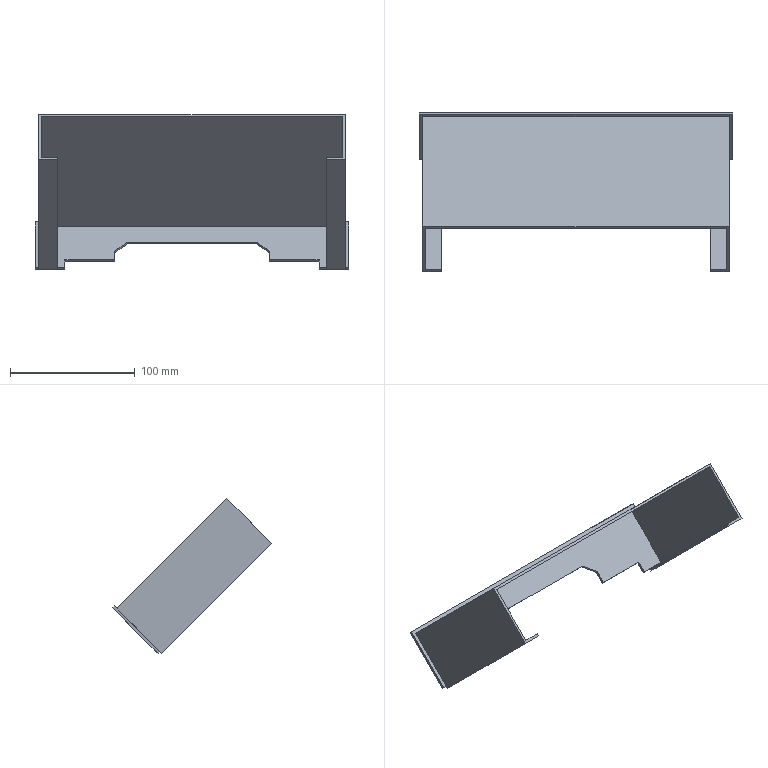Component | SolidWorks | Section3-1 | 2 solids | 30 faces | box 252 x 127.99 x 124.45 mm | volume 110276 mm3 | plane 30
build123d program:
from build123d import *

# Parameters (mm, degrees)
EXTRUDE_THIN1_DEPTH = 125
BOSS_EXTRUDE1_DEPTH = 2


with BuildPart() as part:
    # Sketch1 → Extrude-Thin1 (new body)
    with BuildSketch(Plane.XY):
        Polygon((-42.5, -44), (-57.5, -44), (-57.5, 7), (188.5, 7), (188.5, -44), (173.5, -44), (173.5, -42), (186.5, -42), (186.5, 5), (-55.5, 5), (-55.5, -42), (-42.5, -42), align=None)
    extrude(amount=EXTRUDE_THIN1_DEPTH)


with BuildPart() as body_2:
    # Sketch3 → Boss-Extrude1 (new body)
    with BuildSketch(Plane(origin=(0, 0, 0), x_dir=(-1, 0, 0), z_dir=(0, 0, -1))):
        Polygon((-167.5, -42), (-191.5, -42), (-191.5, 10), (60.5, 10), (60.5, -42), (36.5, -42), (36.5, -33), (-3.5, -33), (-3.5, -23), (-13.5, -13), (-117.5, -13), (-127.5, -23), (-127.5, -33), (-167.5, -33), align=None)
    extrude(amount=BOSS_EXTRUDE1_DEPTH)


solid = Compound([part.part, body_2.part])

# Placed as in the assembly
solid = solid.moved(Location((53.324, -324.22, 131.269), (45, 0, 0)))
STEP:
#1=COLOUR_RGB('',0.7922,0.8196,0.9333);
#2=FILL_AREA_STYLE_COLOUR('',#1);
#3=FILL_AREA_STYLE('',(#2));
#4=SURFACE_STYLE_FILL_AREA(#3);
#5=SURFACE_SIDE_STYLE('',(#4));
#6=SURFACE_STYLE_USAGE(.BOTH.,#5);
#7=PRESENTATION_STYLE_ASSIGNMENT((#6));
#8=CARTESIAN_POINT('',(8.694,-13.934,3.999));
#9=VERTEX_POINT('',#8);
#10=CARTESIAN_POINT('',(8.694,-13.683,4.249));
#11=VERTEX_POINT('',#10);
#12=CARTESIAN_POINT('',(8.694,-13.683,4.249));
#13=DIRECTION('',(-0.,0.7071,0.7071));
#14=VECTOR('',#13,39.37);
#15=LINE('',#12,#14);
#16=EDGE_CURVE('',#9,#11,#15,.T.);
#17=ORIENTED_EDGE('',*,*,#16,.T.);
#18=CARTESIAN_POINT('',(8.694,-13.628,4.194));
#19=VERTEX_POINT('',#18);
#20=CARTESIAN_POINT('',(8.694,-13.628,4.194));
#21=DIRECTION('',(0.,-0.7071,0.7071));
#22=VECTOR('',#21,39.37);
#23=LINE('',#20,#22);
#24=EDGE_CURVE('',#19,#11,#23,.T.);
#25=ORIENTED_EDGE('',*,*,#24,.F.);
#26=CARTESIAN_POINT('',(8.694,-13.878,3.943));
#27=VERTEX_POINT('',#26);
#28=CARTESIAN_POINT('',(8.694,-13.628,4.194));
#29=DIRECTION('',(-0.,0.7071,0.7071));
#30=VECTOR('',#29,39.37);
#31=LINE('',#28,#30);
#32=EDGE_CURVE('',#27,#19,#31,.T.);
#33=ORIENTED_EDGE('',*,*,#32,.F.);
#34=CARTESIAN_POINT('',(8.694,-13.878,3.943));
#35=DIRECTION('',(0.,-0.7071,0.7071));
#36=VECTOR('',#35,39.37);
#37=LINE('',#34,#36);
#38=EDGE_CURVE('',#27,#9,#37,.T.);
#39=ORIENTED_EDGE('',*,*,#38,.T.);
#40=EDGE_LOOP('',(#17,#25,#33,#39));
#41=FACE_OUTER_BOUND('',#40,.T.);
#42=CARTESIAN_POINT('',(8.694,-13.628,4.194));
#43=DIRECTION('',(1.,0.,-0.));
#44=DIRECTION('',(-0.,0.7071,-0.7071));
#45=AXIS2_PLACEMENT_3D('',#42,#43,#44);
#46=PLANE('',#45);
#47=ADVANCED_FACE('',(#41),#46,.F.);
#48=CARTESIAN_POINT('',(7.119,-13.683,4.249));
#49=VERTEX_POINT('',#48);
#50=CARTESIAN_POINT('',(7.119,-13.683,4.249));
#51=DIRECTION('',(-1.,-0.,0.));
#52=VECTOR('',#51,39.37);
#53=LINE('',#50,#52);
#54=EDGE_CURVE('',#11,#49,#53,.T.);
#55=ORIENTED_EDGE('',*,*,#54,.T.);
#56=CARTESIAN_POINT('',(7.119,-13.628,4.194));
#57=VERTEX_POINT('',#56);
#58=CARTESIAN_POINT('',(7.119,-13.628,4.194));
#59=DIRECTION('',(0.,-0.7071,0.7071));
#60=VECTOR('',#59,39.37);
#61=LINE('',#58,#60);
#62=EDGE_CURVE('',#57,#49,#61,.T.);
#63=ORIENTED_EDGE('',*,*,#62,.F.);
#64=CARTESIAN_POINT('',(7.119,-13.628,4.194));
#65=DIRECTION('',(-1.,-0.,0.));
#66=VECTOR('',#65,39.37);
#67=LINE('',#64,#66);
#68=EDGE_CURVE('',#19,#57,#67,.T.);
#69=ORIENTED_EDGE('',*,*,#68,.F.);
#70=ORIENTED_EDGE('',*,*,#24,.T.);
#71=EDGE_LOOP('',(#55,#63,#69,#70));
#72=FACE_OUTER_BOUND('',#71,.T.);
#73=CARTESIAN_POINT('',(7.119,-13.628,4.194));
#74=DIRECTION('',(-0.,0.7071,0.7071));
#75=DIRECTION('',(0.,-0.7071,0.7071));
#76=AXIS2_PLACEMENT_3D('',#73,#74,#75);
#77=PLANE('',#76);
#78=ADVANCED_FACE('',(#72),#77,.F.);
#79=CARTESIAN_POINT('',(7.119,-13.405,4.528));
#80=VERTEX_POINT('',#79);
#81=CARTESIAN_POINT('',(7.119,-13.405,4.528));
#82=DIRECTION('',(0.,0.7071,0.7071));
#83=VECTOR('',#82,39.37);
#84=LINE('',#81,#83);
#85=EDGE_CURVE('',#49,#80,#84,.T.);
#86=ORIENTED_EDGE('',*,*,#85,.T.);
#87=CARTESIAN_POINT('',(7.119,-13.349,4.472));
#88=VERTEX_POINT('',#87);
#89=CARTESIAN_POINT('',(7.119,-13.349,4.472));
#90=DIRECTION('',(0.,-0.7071,0.7071));
#91=VECTOR('',#90,39.37);
#92=LINE('',#89,#91);
#93=EDGE_CURVE('',#88,#80,#92,.T.);
#94=ORIENTED_EDGE('',*,*,#93,.F.);
#95=CARTESIAN_POINT('',(7.119,-13.349,4.472));
#96=DIRECTION('',(0.,0.7071,0.7071));
#97=VECTOR('',#96,39.37);
#98=LINE('',#95,#97);
#99=EDGE_CURVE('',#57,#88,#98,.T.);
#100=ORIENTED_EDGE('',*,*,#99,.F.);
#101=ORIENTED_EDGE('',*,*,#62,.T.);
#102=EDGE_LOOP('',(#86,#94,#100,#101));
#103=FACE_OUTER_BOUND('',#102,.T.);
#104=CARTESIAN_POINT('',(7.119,-13.349,4.472));
#105=DIRECTION('',(1.,-0.,-0.));
#106=DIRECTION('',(0.,0.7071,0.7071));
#107=AXIS2_PLACEMENT_3D('',#104,#105,#106);
#108=PLANE('',#107);
#109=ADVANCED_FACE('',(#103),#108,.F.);
#110=CARTESIAN_POINT('',(6.725,-13.126,4.806));
#111=VERTEX_POINT('',#110);
#112=CARTESIAN_POINT('',(6.725,-13.126,4.806));
#113=DIRECTION('',(-0.7071,0.5,0.5));
#114=VECTOR('',#113,39.37);
#115=LINE('',#112,#114);
#116=EDGE_CURVE('',#80,#111,#115,.T.);
#117=ORIENTED_EDGE('',*,*,#116,.T.);
#118=CARTESIAN_POINT('',(6.725,-13.071,4.751));
#119=VERTEX_POINT('',#118);
#120=CARTESIAN_POINT('',(6.725,-13.071,4.751));
#121=DIRECTION('',(0.,-0.7071,0.7071));
#122=VECTOR('',#121,39.37);
#123=LINE('',#120,#122);
#124=EDGE_CURVE('',#119,#111,#123,.T.);
#125=ORIENTED_EDGE('',*,*,#124,.F.);
#126=CARTESIAN_POINT('',(6.725,-13.071,4.751));
#127=DIRECTION('',(-0.7071,0.5,0.5));
#128=VECTOR('',#127,39.37);
#129=LINE('',#126,#128);
#130=EDGE_CURVE('',#88,#119,#129,.T.);
#131=ORIENTED_EDGE('',*,*,#130,.F.);
#132=ORIENTED_EDGE('',*,*,#93,.T.);
#133=EDGE_LOOP('',(#117,#125,#131,#132));
#134=FACE_OUTER_BOUND('',#133,.T.);
#135=CARTESIAN_POINT('',(6.725,-13.071,4.751));
#136=DIRECTION('',(0.7071,0.5,0.5));
#137=DIRECTION('',(-0.7071,0.5,0.5));
#138=AXIS2_PLACEMENT_3D('',#135,#136,#137);
#139=PLANE('',#138);
#140=ADVANCED_FACE('',(#134),#139,.F.);
#141=CARTESIAN_POINT('',(2.631,-13.126,4.806));
#142=VERTEX_POINT('',#141);
#143=CARTESIAN_POINT('',(2.631,-13.126,4.806));
#144=DIRECTION('',(-1.,-0.,0.));
#145=VECTOR('',#144,39.37);
#146=LINE('',#143,#145);
#147=EDGE_CURVE('',#111,#142,#146,.T.);
#148=ORIENTED_EDGE('',*,*,#147,.T.);
#149=CARTESIAN_POINT('',(2.631,-13.071,4.751));
#150=VERTEX_POINT('',#149);
#151=CARTESIAN_POINT('',(2.631,-13.071,4.751));
#152=DIRECTION('',(0.,-0.7071,0.7071));
#153=VECTOR('',#152,39.37);
#154=LINE('',#151,#153);
#155=EDGE_CURVE('',#150,#142,#154,.T.);
#156=ORIENTED_EDGE('',*,*,#155,.F.);
#157=CARTESIAN_POINT('',(2.631,-13.071,4.751));
#158=DIRECTION('',(-1.,-0.,0.));
#159=VECTOR('',#158,39.37);
#160=LINE('',#157,#159);
#161=EDGE_CURVE('',#119,#150,#160,.T.);
#162=ORIENTED_EDGE('',*,*,#161,.F.);
#163=ORIENTED_EDGE('',*,*,#124,.T.);
#164=EDGE_LOOP('',(#148,#156,#162,#163));
#165=FACE_OUTER_BOUND('',#164,.T.);
#166=CARTESIAN_POINT('',(2.631,-13.071,4.751));
#167=DIRECTION('',(0.,0.7071,0.7071));
#168=DIRECTION('',(-1.,-0.,0.));
#169=AXIS2_PLACEMENT_3D('',#166,#167,#168);
#170=PLANE('',#169);
#171=ADVANCED_FACE('',(#165),#170,.F.);
#172=CARTESIAN_POINT('',(2.237,-13.405,4.528));
#173=VERTEX_POINT('',#172);
#174=CARTESIAN_POINT('',(2.237,-13.405,4.528));
#175=DIRECTION('',(-0.7071,-0.5,-0.5));
#176=VECTOR('',#175,39.37);
#177=LINE('',#174,#176);
#178=EDGE_CURVE('',#142,#173,#177,.T.);
#179=ORIENTED_EDGE('',*,*,#178,.T.);
#180=CARTESIAN_POINT('',(2.237,-13.349,4.472));
#181=VERTEX_POINT('',#180);
#182=CARTESIAN_POINT('',(2.237,-13.349,4.472));
#183=DIRECTION('',(0.,-0.7071,0.7071));
#184=VECTOR('',#183,39.37);
#185=LINE('',#182,#184);
#186=EDGE_CURVE('',#181,#173,#185,.T.);
#187=ORIENTED_EDGE('',*,*,#186,.F.);
#188=CARTESIAN_POINT('',(2.237,-13.349,4.472));
#189=DIRECTION('',(-0.7071,-0.5,-0.5));
#190=VECTOR('',#189,39.37);
#191=LINE('',#188,#190);
#192=EDGE_CURVE('',#150,#181,#191,.T.);
#193=ORIENTED_EDGE('',*,*,#192,.F.);
#194=ORIENTED_EDGE('',*,*,#155,.T.);
#195=EDGE_LOOP('',(#179,#187,#193,#194));
#196=FACE_OUTER_BOUND('',#195,.T.);
#197=CARTESIAN_POINT('',(2.237,-13.349,4.472));
#198=DIRECTION('',(-0.7071,0.5,0.5));
#199=DIRECTION('',(-0.7071,-0.5,-0.5));
#200=AXIS2_PLACEMENT_3D('',#197,#198,#199);
#201=PLANE('',#200);
#202=ADVANCED_FACE('',(#196),#201,.F.);
#203=CARTESIAN_POINT('',(2.237,-13.683,4.249));
#204=VERTEX_POINT('',#203);
#205=CARTESIAN_POINT('',(2.237,-13.683,4.249));
#206=DIRECTION('',(-0.,-0.7071,-0.7071));
#207=VECTOR('',#206,39.37);
#208=LINE('',#205,#207);
#209=EDGE_CURVE('',#173,#204,#208,.T.);
#210=ORIENTED_EDGE('',*,*,#209,.T.);
#211=CARTESIAN_POINT('',(2.237,-13.628,4.194));
#212=VERTEX_POINT('',#211);
#213=CARTESIAN_POINT('',(2.237,-13.628,4.194));
#214=DIRECTION('',(0.,-0.7071,0.7071));
#215=VECTOR('',#214,39.37);
#216=LINE('',#213,#215);
#217=EDGE_CURVE('',#212,#204,#216,.T.);
#218=ORIENTED_EDGE('',*,*,#217,.F.);
#219=CARTESIAN_POINT('',(2.237,-13.628,4.194));
#220=DIRECTION('',(-0.,-0.7071,-0.7071));
#221=VECTOR('',#220,39.37);
#222=LINE('',#219,#221);
#223=EDGE_CURVE('',#181,#212,#222,.T.);
#224=ORIENTED_EDGE('',*,*,#223,.F.);
#225=ORIENTED_EDGE('',*,*,#186,.T.);
#226=EDGE_LOOP('',(#210,#218,#224,#225));
#227=FACE_OUTER_BOUND('',#226,.T.);
#228=CARTESIAN_POINT('',(2.237,-13.628,4.194));
#229=DIRECTION('',(-1.,0.,0.));
#230=DIRECTION('',(-0.,-0.7071,-0.7071));
#231=AXIS2_PLACEMENT_3D('',#228,#229,#230);
#232=PLANE('',#231);
#233=ADVANCED_FACE('',(#227),#232,.F.);
#234=CARTESIAN_POINT('',(0.6624,-13.683,4.249));
#235=VERTEX_POINT('',#234);
#236=CARTESIAN_POINT('',(0.6624,-13.683,4.249));
#237=DIRECTION('',(-1.,-0.,0.));
#238=VECTOR('',#237,39.37);
#239=LINE('',#236,#238);
#240=EDGE_CURVE('',#204,#235,#239,.T.);
#241=ORIENTED_EDGE('',*,*,#240,.T.);
#242=CARTESIAN_POINT('',(0.6624,-13.628,4.194));
#243=VERTEX_POINT('',#242);
#244=CARTESIAN_POINT('',(0.6624,-13.628,4.194));
#245=DIRECTION('',(0.,-0.7071,0.7071));
#246=VECTOR('',#245,39.37);
#247=LINE('',#244,#246);
#248=EDGE_CURVE('',#243,#235,#247,.T.);
#249=ORIENTED_EDGE('',*,*,#248,.F.);
#250=CARTESIAN_POINT('',(0.6624,-13.628,4.194));
#251=DIRECTION('',(-1.,-0.,0.));
#252=VECTOR('',#251,39.37);
#253=LINE('',#250,#252);
#254=EDGE_CURVE('',#212,#243,#253,.T.);
#255=ORIENTED_EDGE('',*,*,#254,.F.);
#256=ORIENTED_EDGE('',*,*,#217,.T.);
#257=EDGE_LOOP('',(#241,#249,#255,#256));
#258=FACE_OUTER_BOUND('',#257,.T.);
#259=CARTESIAN_POINT('',(0.6624,-13.628,4.194));
#260=DIRECTION('',(0.,0.7071,0.7071));
#261=DIRECTION('',(-1.,-0.,0.));
#262=AXIS2_PLACEMENT_3D('',#259,#260,#261);
#263=PLANE('',#262);
#264=ADVANCED_FACE('',(#258),#263,.F.);
#265=CARTESIAN_POINT('',(0.6624,-13.934,3.999));
#266=VERTEX_POINT('',#265);
#267=CARTESIAN_POINT('',(0.6624,-13.934,3.999));
#268=DIRECTION('',(0.,-0.7071,-0.7071));
#269=VECTOR('',#268,39.37);
#270=LINE('',#267,#269);
#271=EDGE_CURVE('',#235,#266,#270,.T.);
#272=ORIENTED_EDGE('',*,*,#271,.T.);
#273=CARTESIAN_POINT('',(0.6624,-13.878,3.943));
#274=VERTEX_POINT('',#273);
#275=CARTESIAN_POINT('',(0.6624,-13.878,3.943));
#276=DIRECTION('',(0.,-0.7071,0.7071));
#277=VECTOR('',#276,39.37);
#278=LINE('',#275,#277);
#279=EDGE_CURVE('',#274,#266,#278,.T.);
#280=ORIENTED_EDGE('',*,*,#279,.F.);
#281=CARTESIAN_POINT('',(0.6624,-13.878,3.943));
#282=DIRECTION('',(0.,-0.7071,-0.7071));
#283=VECTOR('',#282,39.37);
#284=LINE('',#281,#283);
#285=EDGE_CURVE('',#243,#274,#284,.T.);
#286=ORIENTED_EDGE('',*,*,#285,.F.);
#287=ORIENTED_EDGE('',*,*,#248,.T.);
#288=EDGE_LOOP('',(#272,#280,#286,#287));
#289=FACE_OUTER_BOUND('',#288,.T.);
#290=CARTESIAN_POINT('',(0.6624,-13.878,3.943));
#291=DIRECTION('',(-1.,-0.,0.));
#292=DIRECTION('',(0.,-0.7071,0.7071));
#293=AXIS2_PLACEMENT_3D('',#290,#291,#292);
#294=PLANE('',#293);
#295=ADVANCED_FACE('',(#289),#294,.F.);
#296=CARTESIAN_POINT('',(-0.2825,-13.934,3.999));
#297=VERTEX_POINT('',#296);
#298=CARTESIAN_POINT('',(-0.2825,-13.934,3.999));
#299=DIRECTION('',(-1.,-0.,0.));
#300=VECTOR('',#299,39.37);
#301=LINE('',#298,#300);
#302=EDGE_CURVE('',#266,#297,#301,.T.);
#303=ORIENTED_EDGE('',*,*,#302,.T.);
#304=CARTESIAN_POINT('',(-0.2825,-13.878,3.943));
#305=VERTEX_POINT('',#304);
#306=CARTESIAN_POINT('',(-0.2825,-13.878,3.943));
#307=DIRECTION('',(0.,-0.7071,0.7071));
#308=VECTOR('',#307,39.37);
#309=LINE('',#306,#308);
#310=EDGE_CURVE('',#305,#297,#309,.T.);
#311=ORIENTED_EDGE('',*,*,#310,.F.);
#312=CARTESIAN_POINT('',(-0.2825,-13.878,3.943));
#313=DIRECTION('',(-1.,-0.,0.));
#314=VECTOR('',#313,39.37);
#315=LINE('',#312,#314);
#316=EDGE_CURVE('',#274,#305,#315,.T.);
#317=ORIENTED_EDGE('',*,*,#316,.F.);
#318=ORIENTED_EDGE('',*,*,#279,.T.);
#319=EDGE_LOOP('',(#303,#311,#317,#318));
#320=FACE_OUTER_BOUND('',#319,.T.);
#321=CARTESIAN_POINT('',(-0.2825,-13.878,3.943));
#322=DIRECTION('',(-0.,0.7071,0.7071));
#323=DIRECTION('',(0.,-0.7071,0.7071));
#324=AXIS2_PLACEMENT_3D('',#321,#322,#323);
#325=PLANE('',#324);
#326=ADVANCED_FACE('',(#320),#325,.F.);
#327=CARTESIAN_POINT('',(-0.2825,-12.486,5.446));
#328=VERTEX_POINT('',#327);
#329=CARTESIAN_POINT('',(-0.2825,-12.486,5.446));
#330=DIRECTION('',(0.,0.7071,0.7071));
#331=VECTOR('',#330,39.37);
#332=LINE('',#329,#331);
#333=EDGE_CURVE('',#297,#328,#332,.T.);
#334=ORIENTED_EDGE('',*,*,#333,.T.);
#335=CARTESIAN_POINT('',(-0.2825,-12.431,5.391));
#336=VERTEX_POINT('',#335);
#337=CARTESIAN_POINT('',(-0.2825,-12.431,5.391));
#338=DIRECTION('',(0.,-0.7071,0.7071));
#339=VECTOR('',#338,39.37);
#340=LINE('',#337,#339);
#341=EDGE_CURVE('',#336,#328,#340,.T.);
#342=ORIENTED_EDGE('',*,*,#341,.F.);
#343=CARTESIAN_POINT('',(-0.2825,-12.431,5.391));
#344=DIRECTION('',(0.,0.7071,0.7071));
#345=VECTOR('',#344,39.37);
#346=LINE('',#343,#345);
#347=EDGE_CURVE('',#305,#336,#346,.T.);
#348=ORIENTED_EDGE('',*,*,#347,.F.);
#349=ORIENTED_EDGE('',*,*,#310,.T.);
#350=EDGE_LOOP('',(#334,#342,#348,#349));
#351=FACE_OUTER_BOUND('',#350,.T.);
#352=CARTESIAN_POINT('',(-0.2825,-12.431,5.391));
#353=DIRECTION('',(1.,0.,-0.));
#354=DIRECTION('',(0.,0.7071,0.7071));
#355=AXIS2_PLACEMENT_3D('',#352,#353,#354);
#356=PLANE('',#355);
#357=ADVANCED_FACE('',(#351),#356,.F.);
#358=CARTESIAN_POINT('',(9.639,-12.486,5.446));
#359=VERTEX_POINT('',#358);
#360=CARTESIAN_POINT('',(9.639,-12.486,5.446));
#361=DIRECTION('',(1.,0.,-0.));
#362=VECTOR('',#361,39.37);
#363=LINE('',#360,#362);
#364=EDGE_CURVE('',#328,#359,#363,.T.);
#365=ORIENTED_EDGE('',*,*,#364,.T.);
#366=CARTESIAN_POINT('',(9.639,-12.431,5.391));
#367=VERTEX_POINT('',#366);
#368=CARTESIAN_POINT('',(9.639,-12.431,5.391));
#369=DIRECTION('',(0.,-0.7071,0.7071));
#370=VECTOR('',#369,39.37);
#371=LINE('',#368,#370);
#372=EDGE_CURVE('',#367,#359,#371,.T.);
#373=ORIENTED_EDGE('',*,*,#372,.F.);
#374=CARTESIAN_POINT('',(9.639,-12.431,5.391));
#375=DIRECTION('',(1.,0.,-0.));
#376=VECTOR('',#375,39.37);
#377=LINE('',#374,#376);
#378=EDGE_CURVE('',#336,#367,#377,.T.);
#379=ORIENTED_EDGE('',*,*,#378,.F.);
#380=ORIENTED_EDGE('',*,*,#341,.T.);
#381=EDGE_LOOP('',(#365,#373,#379,#380));
#382=FACE_OUTER_BOUND('',#381,.T.);
#383=CARTESIAN_POINT('',(9.639,-12.431,5.391));
#384=DIRECTION('',(0.,-0.7071,-0.7071));
#385=DIRECTION('',(-0.,0.7071,-0.7071));
#386=AXIS2_PLACEMENT_3D('',#383,#384,#385);
#387=PLANE('',#386);
#388=ADVANCED_FACE('',(#382),#387,.F.);
#389=CARTESIAN_POINT('',(9.639,-13.934,3.999));
#390=VERTEX_POINT('',#389);
#391=CARTESIAN_POINT('',(9.639,-13.934,3.999));
#392=DIRECTION('',(0.,-0.7071,-0.7071));
#393=VECTOR('',#392,39.37);
#394=LINE('',#391,#393);
#395=EDGE_CURVE('',#359,#390,#394,.T.);
#396=ORIENTED_EDGE('',*,*,#395,.T.);
#397=CARTESIAN_POINT('',(9.639,-13.878,3.943));
#398=VERTEX_POINT('',#397);
#399=CARTESIAN_POINT('',(9.639,-13.878,3.943));
#400=DIRECTION('',(0.,-0.7071,0.7071));
#401=VECTOR('',#400,39.37);
#402=LINE('',#399,#401);
#403=EDGE_CURVE('',#398,#390,#402,.T.);
#404=ORIENTED_EDGE('',*,*,#403,.F.);
#405=CARTESIAN_POINT('',(9.639,-13.878,3.943));
#406=DIRECTION('',(0.,-0.7071,-0.7071));
#407=VECTOR('',#406,39.37);
#408=LINE('',#405,#407);
#409=EDGE_CURVE('',#367,#398,#408,.T.);
#410=ORIENTED_EDGE('',*,*,#409,.F.);
#411=ORIENTED_EDGE('',*,*,#372,.T.);
#412=EDGE_LOOP('',(#396,#404,#410,#411));
#413=FACE_OUTER_BOUND('',#412,.T.);
#414=CARTESIAN_POINT('',(9.639,-13.878,3.943));
#415=DIRECTION('',(-1.,-0.,0.));
#416=DIRECTION('',(0.,-0.7071,0.7071));
#417=AXIS2_PLACEMENT_3D('',#414,#415,#416);
#418=PLANE('',#417);
#419=ADVANCED_FACE('',(#413),#418,.F.);
#420=CARTESIAN_POINT('',(8.694,-13.934,3.999));
#421=DIRECTION('',(-1.,-0.,-0.));
#422=VECTOR('',#421,39.37);
#423=LINE('',#420,#422);
#424=EDGE_CURVE('',#390,#9,#423,.T.);
#425=ORIENTED_EDGE('',*,*,#424,.T.);
#426=ORIENTED_EDGE('',*,*,#38,.F.);
#427=CARTESIAN_POINT('',(8.694,-13.878,3.943));
#428=DIRECTION('',(-1.,-0.,-0.));
#429=VECTOR('',#428,39.37);
#430=LINE('',#427,#429);
#431=EDGE_CURVE('',#398,#27,#430,.T.);
#432=ORIENTED_EDGE('',*,*,#431,.F.);
#433=ORIENTED_EDGE('',*,*,#403,.T.);
#434=EDGE_LOOP('',(#425,#426,#432,#433));
#435=FACE_OUTER_BOUND('',#434,.T.);
#436=CARTESIAN_POINT('',(8.694,-13.878,3.943));
#437=DIRECTION('',(-0.,0.7071,0.7071));
#438=DIRECTION('',(-1.,-0.,-0.));
#439=AXIS2_PLACEMENT_3D('',#436,#437,#438);
#440=PLANE('',#439);
#441=ADVANCED_FACE('',(#435),#440,.F.);
#442=ORIENTED_EDGE('',*,*,#32,.T.);
#443=ORIENTED_EDGE('',*,*,#68,.T.);
#444=ORIENTED_EDGE('',*,*,#99,.T.);
#445=ORIENTED_EDGE('',*,*,#130,.T.);
#446=ORIENTED_EDGE('',*,*,#161,.T.);
#447=ORIENTED_EDGE('',*,*,#192,.T.);
#448=ORIENTED_EDGE('',*,*,#223,.T.);
#449=ORIENTED_EDGE('',*,*,#254,.T.);
#450=ORIENTED_EDGE('',*,*,#285,.T.);
#451=ORIENTED_EDGE('',*,*,#316,.T.);
#452=ORIENTED_EDGE('',*,*,#347,.T.);
#453=ORIENTED_EDGE('',*,*,#378,.T.);
#454=ORIENTED_EDGE('',*,*,#409,.T.);
#455=ORIENTED_EDGE('',*,*,#431,.T.);
#456=EDGE_LOOP('',(#442,#443,#444,#445,#446,#447,#448,#449,#450,#451,#452,#453,#454,#455));
#457=FACE_OUTER_BOUND('',#456,.T.);
#458=CARTESIAN_POINT('',(2.099,-12.709,5.112));
#459=DIRECTION('',(0.,-0.7071,0.7071));
#460=DIRECTION('',(1.,0.,-0.));
#461=AXIS2_PLACEMENT_3D('',#458,#459,#460);
#462=PLANE('',#461);
#463=ADVANCED_FACE('',(#457),#462,.F.);
#464=ORIENTED_EDGE('',*,*,#16,.F.);
#465=ORIENTED_EDGE('',*,*,#424,.F.);
#466=ORIENTED_EDGE('',*,*,#395,.F.);
#467=ORIENTED_EDGE('',*,*,#364,.F.);
#468=ORIENTED_EDGE('',*,*,#333,.F.);
#469=ORIENTED_EDGE('',*,*,#302,.F.);
#470=ORIENTED_EDGE('',*,*,#271,.F.);
#471=ORIENTED_EDGE('',*,*,#240,.F.);
#472=ORIENTED_EDGE('',*,*,#209,.F.);
#473=ORIENTED_EDGE('',*,*,#178,.F.);
#474=ORIENTED_EDGE('',*,*,#147,.F.);
#475=ORIENTED_EDGE('',*,*,#116,.F.);
#476=ORIENTED_EDGE('',*,*,#85,.F.);
#477=ORIENTED_EDGE('',*,*,#54,.F.);
#478=EDGE_LOOP('',(#464,#465,#466,#467,#468,#469,#470,#471,#472,#473,#474,#475,#476,#477));
#479=FACE_OUTER_BOUND('',#478,.T.);
#480=CARTESIAN_POINT('',(2.099,-12.765,5.168));
#481=DIRECTION('',(0.,-0.7071,0.7071));
#482=DIRECTION('',(1.,0.,-0.));
#483=AXIS2_PLACEMENT_3D('',#480,#481,#482);
#484=PLANE('',#483);
#485=ADVANCED_FACE('',(#479),#484,.T.);
#486=CLOSED_SHELL('',(#47,#78,#109,#140,#171,#202,#233,#264,#295,#326,#357,#388,#419,#441,#463,#485));
#487=MANIFOLD_SOLID_BREP('',#486);
#488=STYLED_ITEM('',(#7),#487);
#489=(LENGTH_UNIT()NAMED_UNIT(*)SI_UNIT($,.METRE.));
#490=LENGTH_MEASURE_WITH_UNIT(LENGTH_MEASURE(0.0254),#489);
#491=DIMENSIONAL_EXPONENTS(1.,0.,0.,0.,0.,0.,0.);
#492=(CONVERSION_BASED_UNIT('',#490)LENGTH_UNIT()NAMED_UNIT(#491));
#493=UNCERTAINTY_MEASURE_WITH_UNIT(LENGTH_MEASURE(0.00001),#492,'','');
#494=(NAMED_UNIT(*)PLANE_ANGLE_UNIT()SI_UNIT($,.RADIAN.));
#495=(NAMED_UNIT(*)SI_UNIT($,.STERADIAN.)SOLID_ANGLE_UNIT());
#496=(GEOMETRIC_REPRESENTATION_CONTEXT(3)GLOBAL_UNCERTAINTY_ASSIGNED_CONTEXT((#493))GLOBAL_UNIT_ASSIGNED_CONTEXT((#492,#494,#495))REPRESENTATION_CONTEXT('',''));
#497=MECHANICAL_DESIGN_GEOMETRIC_PRESENTATION_REPRESENTATION('',(#488),#496);
#498=PRESENTATION_LAYER_ASSIGNMENT('','',(#488));
#499=CARTESIAN_POINT('',(9.442,-13.934,3.999));
#500=VERTEX_POINT('',#499);
#501=CARTESIAN_POINT('',(8.93,-13.934,3.999));
#502=VERTEX_POINT('',#501);
#503=CARTESIAN_POINT('',(9.521,-13.934,3.999));
#504=DIRECTION('',(-1.,-0.,-0.));
#505=VECTOR('',#504,39.37);
#506=LINE('',#503,#505);
#507=EDGE_CURVE('',#500,#502,#506,.T.);
#508=ORIENTED_EDGE('',*,*,#507,.T.);
#509=CARTESIAN_POINT('',(8.93,-17.414,7.479));
#510=VERTEX_POINT('',#509);
#511=CARTESIAN_POINT('',(8.93,-17.414,7.479));
#512=DIRECTION('',(-0.,0.7071,-0.7071));
#513=VECTOR('',#512,39.37);
#514=LINE('',#511,#513);
#515=EDGE_CURVE('',#510,#502,#514,.T.);
#516=ORIENTED_EDGE('',*,*,#515,.F.);
#517=CARTESIAN_POINT('',(9.442,-17.414,7.479));
#518=VERTEX_POINT('',#517);
#519=CARTESIAN_POINT('',(9.521,-17.414,7.479));
#520=DIRECTION('',(-1.,-0.,-0.));
#521=VECTOR('',#520,39.37);
#522=LINE('',#519,#521);
#523=EDGE_CURVE('',#518,#510,#522,.T.);
#524=ORIENTED_EDGE('',*,*,#523,.F.);
#525=CARTESIAN_POINT('',(9.442,-17.414,7.479));
#526=DIRECTION('',(-0.,0.7071,-0.7071));
#527=VECTOR('',#526,39.37);
#528=LINE('',#525,#527);
#529=EDGE_CURVE('',#518,#500,#528,.T.);
#530=ORIENTED_EDGE('',*,*,#529,.T.);
#531=EDGE_LOOP('',(#508,#516,#524,#530));
#532=FACE_OUTER_BOUND('',#531,.T.);
#533=CARTESIAN_POINT('',(9.521,-17.414,7.479));
#534=DIRECTION('',(0.,-0.7071,-0.7071));
#535=DIRECTION('',(1.,0.,0.));
#536=AXIS2_PLACEMENT_3D('',#533,#534,#535);
#537=PLANE('',#536);
#538=ADVANCED_FACE('',(#532),#537,.F.);
#539=CARTESIAN_POINT('',(8.93,-13.989,3.943));
#540=VERTEX_POINT('',#539);
#541=CARTESIAN_POINT('',(8.93,-13.989,3.943));
#542=DIRECTION('',(-0.,0.7071,0.7071));
#543=VECTOR('',#542,39.37);
#544=LINE('',#541,#543);
#545=EDGE_CURVE('',#540,#502,#544,.T.);
#546=ORIENTED_EDGE('',*,*,#545,.F.);
#547=CARTESIAN_POINT('',(8.93,-17.469,7.423));
#548=VERTEX_POINT('',#547);
#549=CARTESIAN_POINT('',(8.93,-17.469,7.423));
#550=DIRECTION('',(-0.,0.7071,-0.7071));
#551=VECTOR('',#550,39.37);
#552=LINE('',#549,#551);
#553=EDGE_CURVE('',#548,#540,#552,.T.);
#554=ORIENTED_EDGE('',*,*,#553,.F.);
#555=CARTESIAN_POINT('',(8.93,-17.469,7.423));
#556=DIRECTION('',(-0.,0.7071,0.7071));
#557=VECTOR('',#556,39.37);
#558=LINE('',#555,#557);
#559=EDGE_CURVE('',#548,#510,#558,.T.);
#560=ORIENTED_EDGE('',*,*,#559,.T.);
#561=ORIENTED_EDGE('',*,*,#515,.T.);
#562=EDGE_LOOP('',(#546,#554,#560,#561));
#563=FACE_OUTER_BOUND('',#562,.T.);
#564=CARTESIAN_POINT('',(8.93,-17.469,7.423));
#565=DIRECTION('',(-1.,-0.,0.));
#566=DIRECTION('',(0.,-0.7071,0.7071));
#567=AXIS2_PLACEMENT_3D('',#564,#565,#566);
#568=PLANE('',#567);
#569=ADVANCED_FACE('',(#563),#568,.T.);
#570=CARTESIAN_POINT('',(9.521,-13.989,3.943));
#571=VERTEX_POINT('',#570);
#572=CARTESIAN_POINT('',(9.521,-13.989,3.943));
#573=DIRECTION('',(-1.,-0.,-0.));
#574=VECTOR('',#573,39.37);
#575=LINE('',#572,#574);
#576=EDGE_CURVE('',#571,#540,#575,.T.);
#577=ORIENTED_EDGE('',*,*,#576,.F.);
#578=CARTESIAN_POINT('',(9.521,-17.469,7.423));
#579=VERTEX_POINT('',#578);
#580=CARTESIAN_POINT('',(9.521,-17.469,7.423));
#581=DIRECTION('',(-0.,0.7071,-0.7071));
#582=VECTOR('',#581,39.37);
#583=LINE('',#580,#582);
#584=EDGE_CURVE('',#579,#571,#583,.T.);
#585=ORIENTED_EDGE('',*,*,#584,.F.);
#586=CARTESIAN_POINT('',(9.521,-17.469,7.423));
#587=DIRECTION('',(-1.,-0.,-0.));
#588=VECTOR('',#587,39.37);
#589=LINE('',#586,#588);
#590=EDGE_CURVE('',#579,#548,#589,.T.);
#591=ORIENTED_EDGE('',*,*,#590,.T.);
#592=ORIENTED_EDGE('',*,*,#553,.T.);
#593=EDGE_LOOP('',(#577,#585,#591,#592));
#594=FACE_OUTER_BOUND('',#593,.T.);
#595=CARTESIAN_POINT('',(9.521,-17.469,7.423));
#596=DIRECTION('',(0.,-0.7071,-0.7071));
#597=DIRECTION('',(1.,0.,0.));
#598=AXIS2_PLACEMENT_3D('',#595,#596,#597);
#599=PLANE('',#598);
#600=ADVANCED_FACE('',(#594),#599,.T.);
#601=CARTESIAN_POINT('',(9.521,-12.57,5.363));
#602=VERTEX_POINT('',#601);
#603=CARTESIAN_POINT('',(9.521,-12.57,5.363));
#604=DIRECTION('',(0.,-0.7071,-0.7071));
#605=VECTOR('',#604,39.37);
#606=LINE('',#603,#605);
#607=EDGE_CURVE('',#602,#571,#606,.T.);
#608=ORIENTED_EDGE('',*,*,#607,.F.);
#609=CARTESIAN_POINT('',(9.521,-16.05,8.843));
#610=VERTEX_POINT('',#609);
#611=CARTESIAN_POINT('',(9.521,-16.05,8.843));
#612=DIRECTION('',(-0.,0.7071,-0.7071));
#613=VECTOR('',#612,39.37);
#614=LINE('',#611,#613);
#615=EDGE_CURVE('',#610,#602,#614,.T.);
#616=ORIENTED_EDGE('',*,*,#615,.F.);
#617=CARTESIAN_POINT('',(9.521,-16.05,8.843));
#618=DIRECTION('',(0.,-0.7071,-0.7071));
#619=VECTOR('',#618,39.37);
#620=LINE('',#617,#619);
#621=EDGE_CURVE('',#610,#579,#620,.T.);
#622=ORIENTED_EDGE('',*,*,#621,.T.);
#623=ORIENTED_EDGE('',*,*,#584,.T.);
#624=EDGE_LOOP('',(#608,#616,#622,#623));
#625=FACE_OUTER_BOUND('',#624,.T.);
#626=CARTESIAN_POINT('',(9.521,-16.05,8.843));
#627=DIRECTION('',(1.,0.,0.));
#628=DIRECTION('',(-0.,0.7071,0.7071));
#629=AXIS2_PLACEMENT_3D('',#626,#627,#628);
#630=PLANE('',#629);
#631=ADVANCED_FACE('',(#625),#630,.T.);
#632=CARTESIAN_POINT('',(-0.1644,-12.57,5.363));
#633=VERTEX_POINT('',#632);
#634=CARTESIAN_POINT('',(-0.1644,-12.57,5.363));
#635=DIRECTION('',(1.,0.,-0.));
#636=VECTOR('',#635,39.37);
#637=LINE('',#634,#636);
#638=EDGE_CURVE('',#633,#602,#637,.T.);
#639=ORIENTED_EDGE('',*,*,#638,.F.);
#640=CARTESIAN_POINT('',(-0.1644,-16.05,8.843));
#641=VERTEX_POINT('',#640);
#642=CARTESIAN_POINT('',(-0.1644,-16.05,8.843));
#643=DIRECTION('',(-0.,0.7071,-0.7071));
#644=VECTOR('',#643,39.37);
#645=LINE('',#642,#644);
#646=EDGE_CURVE('',#641,#633,#645,.T.);
#647=ORIENTED_EDGE('',*,*,#646,.F.);
#648=CARTESIAN_POINT('',(-0.1644,-16.05,8.843));
#649=DIRECTION('',(1.,0.,-0.));
#650=VECTOR('',#649,39.37);
#651=LINE('',#648,#650);
#652=EDGE_CURVE('',#641,#610,#651,.T.);
#653=ORIENTED_EDGE('',*,*,#652,.T.);
#654=ORIENTED_EDGE('',*,*,#615,.T.);
#655=EDGE_LOOP('',(#639,#647,#653,#654));
#656=FACE_OUTER_BOUND('',#655,.T.);
#657=CARTESIAN_POINT('',(-0.1644,-16.05,8.843));
#658=DIRECTION('',(-0.,0.7071,0.7071));
#659=DIRECTION('',(0.,-0.7071,0.7071));
#660=AXIS2_PLACEMENT_3D('',#657,#658,#659);
#661=PLANE('',#660);
#662=ADVANCED_FACE('',(#656),#661,.T.);
#663=CARTESIAN_POINT('',(-0.1644,-13.989,3.943));
#664=VERTEX_POINT('',#663);
#665=CARTESIAN_POINT('',(-0.1644,-13.989,3.943));
#666=DIRECTION('',(-0.,0.7071,0.7071));
#667=VECTOR('',#666,39.37);
#668=LINE('',#665,#667);
#669=EDGE_CURVE('',#664,#633,#668,.T.);
#670=ORIENTED_EDGE('',*,*,#669,.F.);
#671=CARTESIAN_POINT('',(-0.1644,-17.469,7.423));
#672=VERTEX_POINT('',#671);
#673=CARTESIAN_POINT('',(-0.1644,-17.469,7.423));
#674=DIRECTION('',(-0.,0.7071,-0.7071));
#675=VECTOR('',#674,39.37);
#676=LINE('',#673,#675);
#677=EDGE_CURVE('',#672,#664,#676,.T.);
#678=ORIENTED_EDGE('',*,*,#677,.F.);
#679=CARTESIAN_POINT('',(-0.1644,-17.469,7.423));
#680=DIRECTION('',(-0.,0.7071,0.7071));
#681=VECTOR('',#680,39.37);
#682=LINE('',#679,#681);
#683=EDGE_CURVE('',#672,#641,#682,.T.);
#684=ORIENTED_EDGE('',*,*,#683,.T.);
#685=ORIENTED_EDGE('',*,*,#646,.T.);
#686=EDGE_LOOP('',(#670,#678,#684,#685));
#687=FACE_OUTER_BOUND('',#686,.T.);
#688=CARTESIAN_POINT('',(-0.1644,-17.469,7.423));
#689=DIRECTION('',(-1.,-0.,0.));
#690=DIRECTION('',(0.,-0.7071,0.7071));
#691=AXIS2_PLACEMENT_3D('',#688,#689,#690);
#692=PLANE('',#691);
#693=ADVANCED_FACE('',(#687),#692,.T.);
#694=CARTESIAN_POINT('',(0.4262,-13.989,3.943));
#695=VERTEX_POINT('',#694);
#696=CARTESIAN_POINT('',(0.4262,-13.989,3.943));
#697=DIRECTION('',(-1.,-0.,0.));
#698=VECTOR('',#697,39.37);
#699=LINE('',#696,#698);
#700=EDGE_CURVE('',#695,#664,#699,.T.);
#701=ORIENTED_EDGE('',*,*,#700,.F.);
#702=CARTESIAN_POINT('',(0.4262,-17.469,7.423));
#703=VERTEX_POINT('',#702);
#704=CARTESIAN_POINT('',(0.4262,-17.469,7.423));
#705=DIRECTION('',(-0.,0.7071,-0.7071));
#706=VECTOR('',#705,39.37);
#707=LINE('',#704,#706);
#708=EDGE_CURVE('',#703,#695,#707,.T.);
#709=ORIENTED_EDGE('',*,*,#708,.F.);
#710=CARTESIAN_POINT('',(0.4262,-17.469,7.423));
#711=DIRECTION('',(-1.,-0.,0.));
#712=VECTOR('',#711,39.37);
#713=LINE('',#710,#712);
#714=EDGE_CURVE('',#703,#672,#713,.T.);
#715=ORIENTED_EDGE('',*,*,#714,.T.);
#716=ORIENTED_EDGE('',*,*,#677,.T.);
#717=EDGE_LOOP('',(#701,#709,#715,#716));
#718=FACE_OUTER_BOUND('',#717,.T.);
#719=CARTESIAN_POINT('',(0.4262,-17.469,7.423));
#720=DIRECTION('',(0.,-0.7071,-0.7071));
#721=DIRECTION('',(-0.,0.7071,-0.7071));
#722=AXIS2_PLACEMENT_3D('',#719,#720,#721);
#723=PLANE('',#722);
#724=ADVANCED_FACE('',(#718),#723,.T.);
#725=CARTESIAN_POINT('',(0.4262,-13.934,3.999));
#726=VERTEX_POINT('',#725);
#727=CARTESIAN_POINT('',(0.4262,-13.934,3.999));
#728=DIRECTION('',(0.,-0.7071,-0.7071));
#729=VECTOR('',#728,39.37);
#730=LINE('',#727,#729);
#731=EDGE_CURVE('',#726,#695,#730,.T.);
#732=ORIENTED_EDGE('',*,*,#731,.F.);
#733=CARTESIAN_POINT('',(0.4262,-17.414,7.479));
#734=VERTEX_POINT('',#733);
#735=CARTESIAN_POINT('',(0.4262,-17.414,7.479));
#736=DIRECTION('',(-0.,0.7071,-0.7071));
#737=VECTOR('',#736,39.37);
#738=LINE('',#735,#737);
#739=EDGE_CURVE('',#734,#726,#738,.T.);
#740=ORIENTED_EDGE('',*,*,#739,.F.);
#741=CARTESIAN_POINT('',(0.4262,-17.414,7.479));
#742=DIRECTION('',(0.,-0.7071,-0.7071));
#743=VECTOR('',#742,39.37);
#744=LINE('',#741,#743);
#745=EDGE_CURVE('',#734,#703,#744,.T.);
#746=ORIENTED_EDGE('',*,*,#745,.T.);
#747=ORIENTED_EDGE('',*,*,#708,.T.);
#748=EDGE_LOOP('',(#732,#740,#746,#747));
#749=FACE_OUTER_BOUND('',#748,.T.);
#750=CARTESIAN_POINT('',(0.4262,-17.414,7.479));
#751=DIRECTION('',(1.,0.,-0.));
#752=DIRECTION('',(-0.,0.7071,-0.7071));
#753=AXIS2_PLACEMENT_3D('',#750,#751,#752);
#754=PLANE('',#753);
#755=ADVANCED_FACE('',(#749),#754,.T.);
#756=CARTESIAN_POINT('',(-0.08565,-13.934,3.999));
#757=VERTEX_POINT('',#756);
#758=CARTESIAN_POINT('',(0.4262,-13.934,3.999));
#759=DIRECTION('',(-1.,-0.,0.));
#760=VECTOR('',#759,39.37);
#761=LINE('',#758,#760);
#762=EDGE_CURVE('',#726,#757,#761,.T.);
#763=ORIENTED_EDGE('',*,*,#762,.T.);
#764=CARTESIAN_POINT('',(-0.08565,-17.414,7.479));
#765=VERTEX_POINT('',#764);
#766=CARTESIAN_POINT('',(-0.08565,-17.414,7.479));
#767=DIRECTION('',(-0.,0.7071,-0.7071));
#768=VECTOR('',#767,39.37);
#769=LINE('',#766,#768);
#770=EDGE_CURVE('',#765,#757,#769,.T.);
#771=ORIENTED_EDGE('',*,*,#770,.F.);
#772=CARTESIAN_POINT('',(0.4262,-17.414,7.479));
#773=DIRECTION('',(-1.,-0.,0.));
#774=VECTOR('',#773,39.37);
#775=LINE('',#772,#774);
#776=EDGE_CURVE('',#734,#765,#775,.T.);
#777=ORIENTED_EDGE('',*,*,#776,.F.);
#778=ORIENTED_EDGE('',*,*,#739,.T.);
#779=EDGE_LOOP('',(#763,#771,#777,#778));
#780=FACE_OUTER_BOUND('',#779,.T.);
#781=CARTESIAN_POINT('',(0.4262,-17.414,7.479));
#782=DIRECTION('',(0.,-0.7071,-0.7071));
#783=DIRECTION('',(-0.,0.7071,-0.7071));
#784=AXIS2_PLACEMENT_3D('',#781,#782,#783);
#785=PLANE('',#784);
#786=ADVANCED_FACE('',(#780),#785,.F.);
#787=CARTESIAN_POINT('',(-0.08565,-12.625,5.307));
#788=VERTEX_POINT('',#787);
#789=CARTESIAN_POINT('',(-0.08565,-13.989,3.943));
#790=DIRECTION('',(-0.,0.7071,0.7071));
#791=VECTOR('',#790,39.37);
#792=LINE('',#789,#791);
#793=EDGE_CURVE('',#757,#788,#792,.T.);
#794=ORIENTED_EDGE('',*,*,#793,.T.);
#795=CARTESIAN_POINT('',(-0.08565,-16.105,8.787));
#796=VERTEX_POINT('',#795);
#797=CARTESIAN_POINT('',(-0.08565,-16.105,8.787));
#798=DIRECTION('',(-0.,0.7071,-0.7071));
#799=VECTOR('',#798,39.37);
#800=LINE('',#797,#799);
#801=EDGE_CURVE('',#796,#788,#800,.T.);
#802=ORIENTED_EDGE('',*,*,#801,.F.);
#803=CARTESIAN_POINT('',(-0.08565,-17.469,7.423));
#804=DIRECTION('',(-0.,0.7071,0.7071));
#805=VECTOR('',#804,39.37);
#806=LINE('',#803,#805);
#807=EDGE_CURVE('',#765,#796,#806,.T.);
#808=ORIENTED_EDGE('',*,*,#807,.F.);
#809=ORIENTED_EDGE('',*,*,#770,.T.);
#810=EDGE_LOOP('',(#794,#802,#808,#809));
#811=FACE_OUTER_BOUND('',#810,.T.);
#812=CARTESIAN_POINT('',(-0.08565,-17.469,7.423));
#813=DIRECTION('',(-1.,-0.,0.));
#814=DIRECTION('',(0.,-0.7071,0.7071));
#815=AXIS2_PLACEMENT_3D('',#812,#813,#814);
#816=PLANE('',#815);
#817=ADVANCED_FACE('',(#811),#816,.F.);
#818=CARTESIAN_POINT('',(9.442,-12.625,5.307));
#819=VERTEX_POINT('',#818);
#820=CARTESIAN_POINT('',(-0.1644,-12.625,5.307));
#821=DIRECTION('',(1.,0.,-0.));
#822=VECTOR('',#821,39.37);
#823=LINE('',#820,#822);
#824=EDGE_CURVE('',#788,#819,#823,.T.);
#825=ORIENTED_EDGE('',*,*,#824,.T.);
#826=CARTESIAN_POINT('',(9.442,-16.105,8.787));
#827=VERTEX_POINT('',#826);
#828=CARTESIAN_POINT('',(9.442,-16.105,8.787));
#829=DIRECTION('',(-0.,0.7071,-0.7071));
#830=VECTOR('',#829,39.37);
#831=LINE('',#828,#830);
#832=EDGE_CURVE('',#827,#819,#831,.T.);
#833=ORIENTED_EDGE('',*,*,#832,.F.);
#834=CARTESIAN_POINT('',(-0.1644,-16.105,8.787));
#835=DIRECTION('',(1.,0.,-0.));
#836=VECTOR('',#835,39.37);
#837=LINE('',#834,#836);
#838=EDGE_CURVE('',#796,#827,#837,.T.);
#839=ORIENTED_EDGE('',*,*,#838,.F.);
#840=ORIENTED_EDGE('',*,*,#801,.T.);
#841=EDGE_LOOP('',(#825,#833,#839,#840));
#842=FACE_OUTER_BOUND('',#841,.T.);
#843=CARTESIAN_POINT('',(-0.1644,-16.105,8.787));
#844=DIRECTION('',(-0.,0.7071,0.7071));
#845=DIRECTION('',(0.,-0.7071,0.7071));
#846=AXIS2_PLACEMENT_3D('',#843,#844,#845);
#847=PLANE('',#846);
#848=ADVANCED_FACE('',(#842),#847,.F.);
#849=CARTESIAN_POINT('',(9.442,-12.57,5.363));
#850=DIRECTION('',(0.,-0.7071,-0.7071));
#851=VECTOR('',#850,39.37);
#852=LINE('',#849,#851);
#853=EDGE_CURVE('',#819,#500,#852,.T.);
#854=ORIENTED_EDGE('',*,*,#853,.T.);
#855=ORIENTED_EDGE('',*,*,#529,.F.);
#856=CARTESIAN_POINT('',(9.442,-16.05,8.843));
#857=DIRECTION('',(0.,-0.7071,-0.7071));
#858=VECTOR('',#857,39.37);
#859=LINE('',#856,#858);
#860=EDGE_CURVE('',#827,#518,#859,.T.);
#861=ORIENTED_EDGE('',*,*,#860,.F.);
#862=ORIENTED_EDGE('',*,*,#832,.T.);
#863=EDGE_LOOP('',(#854,#855,#861,#862));
#864=FACE_OUTER_BOUND('',#863,.T.);
#865=CARTESIAN_POINT('',(9.442,-16.05,8.843));
#866=DIRECTION('',(1.,0.,0.));
#867=DIRECTION('',(-0.,0.7071,0.7071));
#868=AXIS2_PLACEMENT_3D('',#865,#866,#867);
#869=PLANE('',#868);
#870=ADVANCED_FACE('',(#864),#869,.F.);
#871=ORIENTED_EDGE('',*,*,#523,.T.);
#872=ORIENTED_EDGE('',*,*,#559,.F.);
#873=ORIENTED_EDGE('',*,*,#590,.F.);
#874=ORIENTED_EDGE('',*,*,#621,.F.);
#875=ORIENTED_EDGE('',*,*,#652,.F.);
#876=ORIENTED_EDGE('',*,*,#683,.F.);
#877=ORIENTED_EDGE('',*,*,#714,.F.);
#878=ORIENTED_EDGE('',*,*,#745,.F.);
#879=ORIENTED_EDGE('',*,*,#776,.T.);
#880=ORIENTED_EDGE('',*,*,#807,.T.);
#881=ORIENTED_EDGE('',*,*,#838,.T.);
#882=ORIENTED_EDGE('',*,*,#860,.T.);
#883=EDGE_LOOP('',(#871,#872,#873,#874,#875,#876,#877,#878,#879,#880,#881,#882));
#884=FACE_OUTER_BOUND('',#883,.T.);
#885=CARTESIAN_POINT('',(2.099,-16.244,8.648));
#886=DIRECTION('',(-0.,0.7071,-0.7071));
#887=DIRECTION('',(-1.,-0.,0.));
#888=AXIS2_PLACEMENT_3D('',#885,#886,#887);
#889=PLANE('',#888);
#890=ADVANCED_FACE('',(#884),#889,.F.);
#891=ORIENTED_EDGE('',*,*,#507,.F.);
#892=ORIENTED_EDGE('',*,*,#853,.F.);
#893=ORIENTED_EDGE('',*,*,#824,.F.);
#894=ORIENTED_EDGE('',*,*,#793,.F.);
#895=ORIENTED_EDGE('',*,*,#762,.F.);
#896=ORIENTED_EDGE('',*,*,#731,.T.);
#897=ORIENTED_EDGE('',*,*,#700,.T.);
#898=ORIENTED_EDGE('',*,*,#669,.T.);
#899=ORIENTED_EDGE('',*,*,#638,.T.);
#900=ORIENTED_EDGE('',*,*,#607,.T.);
#901=ORIENTED_EDGE('',*,*,#576,.T.);
#902=ORIENTED_EDGE('',*,*,#545,.T.);
#903=EDGE_LOOP('',(#891,#892,#893,#894,#895,#896,#897,#898,#899,#900,#901,#902));
#904=FACE_OUTER_BOUND('',#903,.T.);
#905=CARTESIAN_POINT('',(2.099,-12.765,5.168));
#906=DIRECTION('',(-0.,0.7071,-0.7071));
#907=DIRECTION('',(-1.,-0.,0.));
#908=AXIS2_PLACEMENT_3D('',#905,#906,#907);
#909=PLANE('',#908);
#910=ADVANCED_FACE('',(#904),#909,.T.);
#911=CLOSED_SHELL('',(#538,#569,#600,#631,#662,#693,#724,#755,#786,#817,#848,#870,#890,#910));
#912=MANIFOLD_SOLID_BREP('',#911);
#913=CARTESIAN_POINT('',(0.,0.,0.));
#914=DIRECTION('',(0.,0.,1.));
#915=DIRECTION('',(1.,0.,0.));
#916=AXIS2_PLACEMENT_3D('',#913,#914,#915);
#917=(LENGTH_UNIT()NAMED_UNIT(*)SI_UNIT($,.METRE.));
#918=LENGTH_MEASURE_WITH_UNIT(LENGTH_MEASURE(0.0254),#917);
#919=DIMENSIONAL_EXPONENTS(1.,0.,0.,0.,0.,0.,0.);
#920=(CONVERSION_BASED_UNIT('',#918)LENGTH_UNIT()NAMED_UNIT(#919));
#921=UNCERTAINTY_MEASURE_WITH_UNIT(LENGTH_MEASURE(0.00001),#920,'','');
#922=(NAMED_UNIT(*)PLANE_ANGLE_UNIT()SI_UNIT($,.RADIAN.));
#923=(NAMED_UNIT(*)SI_UNIT($,.STERADIAN.)SOLID_ANGLE_UNIT());
#924=(GEOMETRIC_REPRESENTATION_CONTEXT(3)GLOBAL_UNCERTAINTY_ASSIGNED_CONTEXT((#921))GLOBAL_UNIT_ASSIGNED_CONTEXT((#920,#922,#923))REPRESENTATION_CONTEXT('',''));
#925=ADVANCED_BREP_SHAPE_REPRESENTATION('',(#487,#912,#916),#924);
#926=COLOUR_RGB('',0.7922,0.8196,0.9333);
#927=FILL_AREA_STYLE_COLOUR('',#926);
#928=FILL_AREA_STYLE('',(#927));
#929=SURFACE_STYLE_FILL_AREA(#928);
#930=SURFACE_SIDE_STYLE('',(#929));
#931=SURFACE_STYLE_USAGE(.BOTH.,#930);
#932=PRESENTATION_STYLE_ASSIGNMENT((#931));
#933=STYLED_ITEM('',(#932),#912);
#934=(LENGTH_UNIT()NAMED_UNIT(*)SI_UNIT($,.METRE.));
#935=LENGTH_MEASURE_WITH_UNIT(LENGTH_MEASURE(0.0254),#934);
#936=DIMENSIONAL_EXPONENTS(1.,0.,0.,0.,0.,0.,0.);
#937=(CONVERSION_BASED_UNIT('',#935)LENGTH_UNIT()NAMED_UNIT(#936));
#938=UNCERTAINTY_MEASURE_WITH_UNIT(LENGTH_MEASURE(0.00001),#937,'','');
#939=(NAMED_UNIT(*)PLANE_ANGLE_UNIT()SI_UNIT($,.RADIAN.));
#940=(NAMED_UNIT(*)SI_UNIT($,.STERADIAN.)SOLID_ANGLE_UNIT());
#941=(GEOMETRIC_REPRESENTATION_CONTEXT(3)GLOBAL_UNCERTAINTY_ASSIGNED_CONTEXT((#938))GLOBAL_UNIT_ASSIGNED_CONTEXT((#937,#939,#940))REPRESENTATION_CONTEXT('',''));
#942=MECHANICAL_DESIGN_GEOMETRIC_PRESENTATION_REPRESENTATION('',(#933),#941);
#943=PRESENTATION_LAYER_ASSIGNMENT('','',(#933));